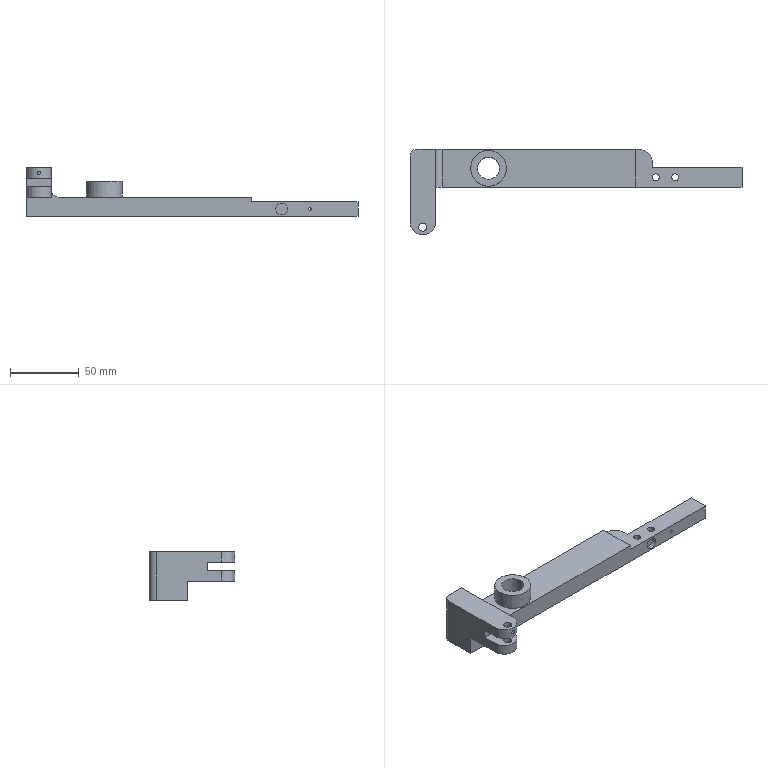Component | SolidWorks | BSH3-03-01Lever-1 | 1 solid | 44 faces | volume 97745 mm3 | cylinder 25 | plane 19 | commonest cylinder face diameters 5 x4 6 x4 2.5 x2 2 x2 8 x2 8.5 x2 16 x2 26 x2